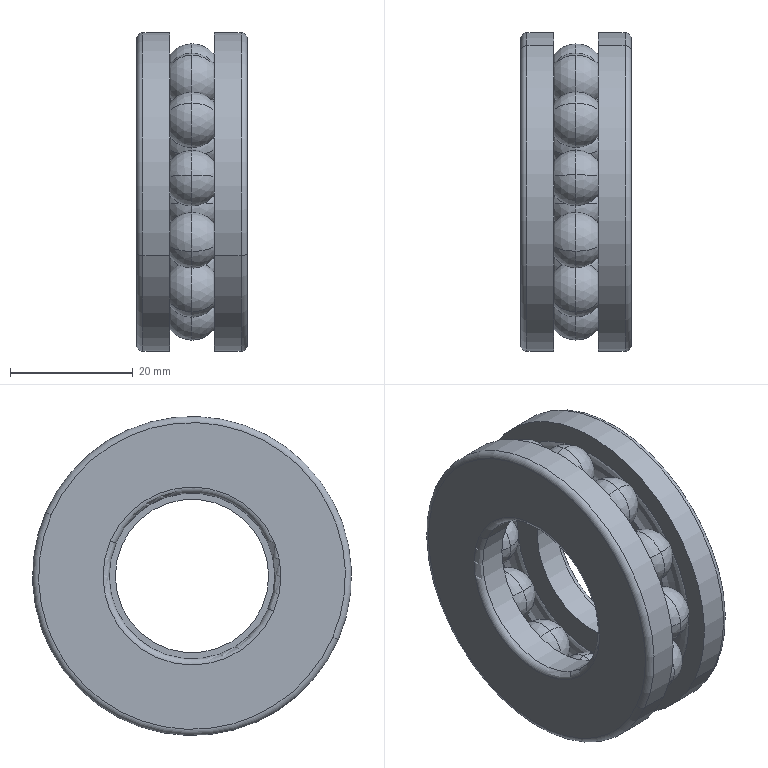Component | SolidWorks | 216InnerTubeAssembly-1_GB_T301-1995[ThrustBallBearing[51000]51305]-1 | 1 solid | 94 faces | volume 20995 mm3 | sphere 48 | torus 32 | cylinder 8 | plane 6 | commonest cylinder face diameters 52 x4 25 x2 27 x2